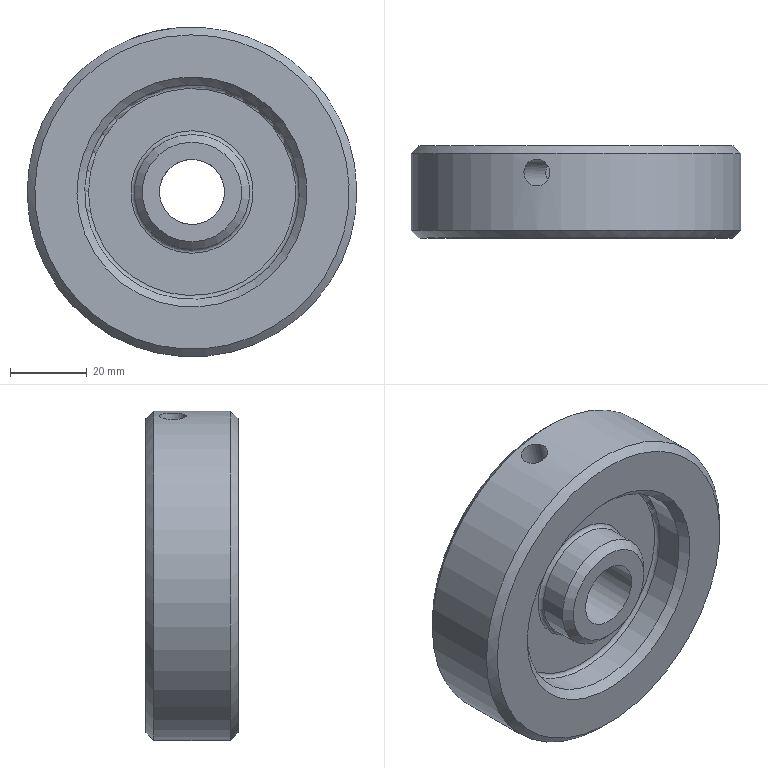Component | NX | FLYWHEEL | 1 solid | 17 faces | volume 113727 mm3 | cylinder 6 | plane 5 | cone 4 | torus 2 | commonest cylinder face diameters 86 x1 17 x1 56 x1 30 x1 5 x1 7 x1